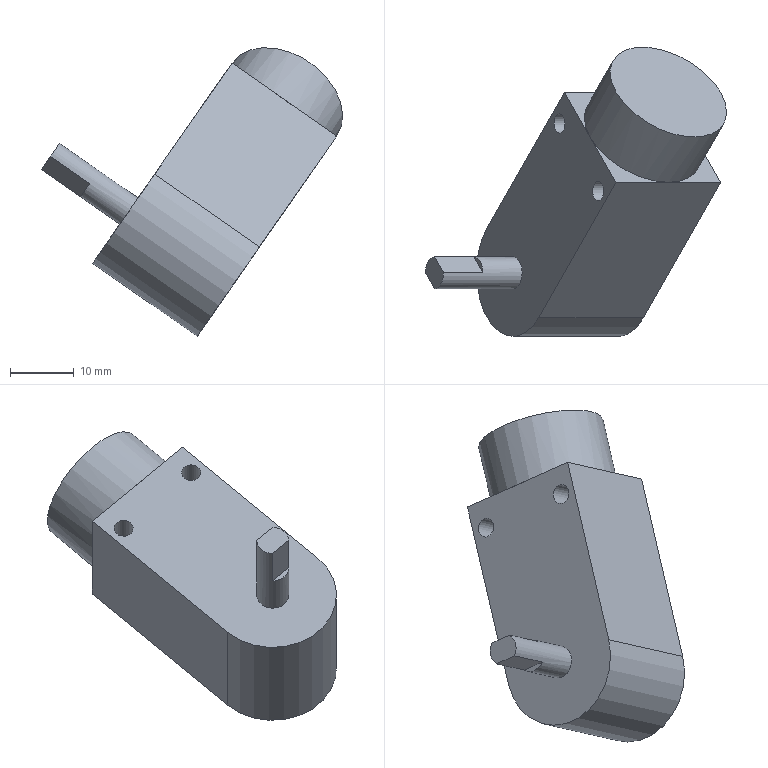Component | NX | MOTOR | 1 solid | 19 faces | volume 18267 mm3 | plane 14 | cylinder 5 | commonest cylinder face diameters 20 x2 3 x2 5 x1